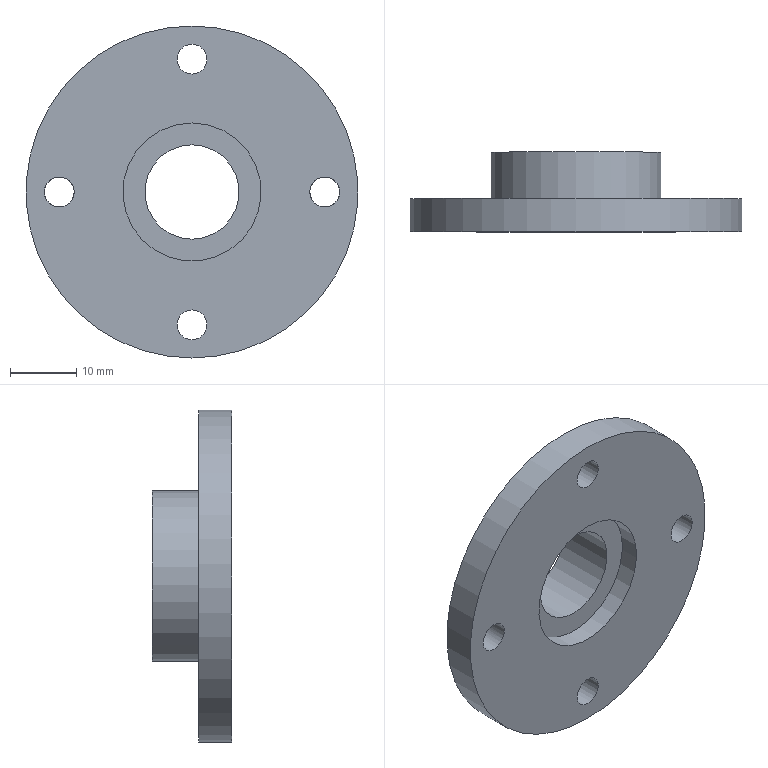Component | NX | END_CAP | 1 solid | 12 faces | box 50 x 12 x 50 mm | volume 10669 mm3 | cylinder 8 | plane 4 | commonest cylinder face diameters 4.5 x4 14.2 x1 20.8 x1 50 x1 25.641 x1
STEP:
#1=CARTESIAN_POINT('',(0.,0.,0.));
#2=DIRECTION('',(0.,0.,1.));
#3=DIRECTION('',(1.,0.,0.));
#4=AXIS2_PLACEMENT_3D('',#1,#2,#3);
#5=CARTESIAN_POINT('',(0.,64.,92.2));
#6=VERTEX_POINT('',#5);
#7=CARTESIAN_POINT('',(0.,64.,85.1));
#8=DIRECTION('',(0.,1.,0.));
#9=DIRECTION('',(0.,0.,1.));
#10=AXIS2_PLACEMENT_3D('',#7,#8,#9);
#11=CIRCLE('',#10,7.1);
#12=CARTESIAN_POINT('',(12.821,64.,85.1));
#13=DIRECTION('',(0.,-1.,0.));
#14=DIRECTION('',(0.,0.,-1.));
#15=AXIS2_PLACEMENT_3D('',#12,#13,#14);
#16=PLANE('',#15);
#17=CARTESIAN_POINT('',(-7.1,-12.821));
#18=CARTESIAN_POINT('',(-7.1,-0.523));
#19=CARTESIAN_POINT('',(3.55,-6.672));
#20=CARTESIAN_POINT('',(14.2,-12.821));
#21=CARTESIAN_POINT('',(3.55,-18.969));
#22=CARTESIAN_POINT('',(-7.1,-25.118));
#23=CARTESIAN_POINT('',(-7.1,-12.821));
#24=(BOUNDED_CURVE()B_SPLINE_CURVE(2,(#17,#18,#19,#20,#21,#22,#23),.UNSPECIFIED.,.T.,.F.)B_SPLINE_CURVE_WITH_KNOTS((1,2,2,2,2,1),(-2.094,0.,2.094,4.189,6.283,8.378),.UNSPECIFIED.)CURVE()GEOMETRIC_REPRESENTATION_ITEM()RATIONAL_B_SPLINE_CURVE((1.,0.5,1.,0.5,1.,0.5,1.))REPRESENTATION_ITEM(''));
#25=(GEOMETRIC_REPRESENTATION_CONTEXT(2)PARAMETRIC_REPRESENTATION_CONTEXT()REPRESENTATION_CONTEXT('',''));
#26=DEFINITIONAL_REPRESENTATION('',(#24),#25);
#27=PCURVE('',#16,#26);
#28=CARTESIAN_POINT('',(0.,52.,85.1));
#29=DIRECTION('',(0.,1.,0.));
#30=DIRECTION('',(0.,0.,1.));
#31=AXIS2_PLACEMENT_3D('',#28,#29,#30);
#32=CYLINDRICAL_SURFACE('',#31,7.1);
#33=CARTESIAN_POINT('',(0.,12.));
#34=DIRECTION('',(1.,0.));
#35=VECTOR('',#34,1.);
#36=LINE('',#33,#35);
#37=(GEOMETRIC_REPRESENTATION_CONTEXT(2)PARAMETRIC_REPRESENTATION_CONTEXT()REPRESENTATION_CONTEXT('',''));
#38=DEFINITIONAL_REPRESENTATION('',(#36),#37);
#39=PCURVE('',#32,#38);
#40=SURFACE_CURVE('',#11,(#27,#39),.PCURVE_S1.);
#41=EDGE_CURVE('',#6,#6,#40,.T.);
#42=ORIENTED_EDGE('',*,*,#41,.F.);
#43=EDGE_LOOP('',(#42));
#44=FACE_BOUND('',#43,.T.);
#45=CARTESIAN_POINT('',(0.,64.,97.921));
#46=VERTEX_POINT('',#45);
#47=CARTESIAN_POINT('',(0.,64.,85.1));
#48=DIRECTION('',(0.,1.,0.));
#49=DIRECTION('',(0.,0.,1.));
#50=AXIS2_PLACEMENT_3D('',#47,#48,#49);
#51=CIRCLE('',#50,12.821);
#52=CARTESIAN_POINT('',(-12.821,-12.821));
#53=CARTESIAN_POINT('',(-12.821,9.385));
#54=CARTESIAN_POINT('',(6.41,-1.718));
#55=CARTESIAN_POINT('',(25.641,-12.821));
#56=CARTESIAN_POINT('',(6.41,-23.923));
#57=CARTESIAN_POINT('',(-12.821,-35.026));
#58=CARTESIAN_POINT('',(-12.821,-12.821));
#59=(BOUNDED_CURVE()B_SPLINE_CURVE(2,(#52,#53,#54,#55,#56,#57,#58),.UNSPECIFIED.,.T.,.F.)B_SPLINE_CURVE_WITH_KNOTS((1,2,2,2,2,1),(-2.094,0.,2.094,4.189,6.283,8.378),.UNSPECIFIED.)CURVE()GEOMETRIC_REPRESENTATION_ITEM()RATIONAL_B_SPLINE_CURVE((1.,0.5,1.,0.5,1.,0.5,1.))REPRESENTATION_ITEM(''));
#60=(GEOMETRIC_REPRESENTATION_CONTEXT(2)PARAMETRIC_REPRESENTATION_CONTEXT()REPRESENTATION_CONTEXT('',''));
#61=DEFINITIONAL_REPRESENTATION('',(#59),#60);
#62=PCURVE('',#16,#61);
#63=CARTESIAN_POINT('',(0.,52.,85.1));
#64=DIRECTION('',(0.,1.,0.));
#65=DIRECTION('',(0.,0.,1.));
#66=AXIS2_PLACEMENT_3D('',#63,#64,#65);
#67=CYLINDRICAL_SURFACE('',#66,12.821);
#68=CARTESIAN_POINT('',(0.,12.));
#69=DIRECTION('',(1.,0.));
#70=VECTOR('',#69,1.);
#71=LINE('',#68,#70);
#72=(GEOMETRIC_REPRESENTATION_CONTEXT(2)PARAMETRIC_REPRESENTATION_CONTEXT()REPRESENTATION_CONTEXT('',''));
#73=DEFINITIONAL_REPRESENTATION('',(#71),#72);
#74=PCURVE('',#67,#73);
#75=SURFACE_CURVE('',#51,(#62,#74),.PCURVE_S1.);
#76=EDGE_CURVE('',#46,#46,#75,.T.);
#77=ORIENTED_EDGE('',*,*,#76,.T.);
#78=EDGE_LOOP('',(#77));
#79=FACE_BOUND('',#78,.T.);
#80=ADVANCED_FACE('',(#44,#79),#16,.F.);
#81=CARTESIAN_POINT('',(0.,55.,92.2));
#82=VERTEX_POINT('',#81);
#83=CARTESIAN_POINT('',(0.,55.,85.1));
#84=DIRECTION('',(0.,1.,0.));
#85=DIRECTION('',(0.,0.,1.));
#86=AXIS2_PLACEMENT_3D('',#83,#84,#85);
#87=CIRCLE('',#86,7.1);
#88=CARTESIAN_POINT('',(0.,3.));
#89=DIRECTION('',(1.,0.));
#90=VECTOR('',#89,1.);
#91=LINE('',#88,#90);
#92=(GEOMETRIC_REPRESENTATION_CONTEXT(2)PARAMETRIC_REPRESENTATION_CONTEXT()REPRESENTATION_CONTEXT('',''));
#93=DEFINITIONAL_REPRESENTATION('',(#91),#92);
#94=PCURVE('',#32,#93);
#95=CARTESIAN_POINT('',(7.1,55.,85.1));
#96=DIRECTION('',(0.,1.,0.));
#97=DIRECTION('',(0.,0.,1.));
#98=AXIS2_PLACEMENT_3D('',#95,#96,#97);
#99=PLANE('',#98);
#100=CARTESIAN_POINT('',(0.,-7.1));
#101=DIRECTION('',(1.,0.));
#102=AXIS2_PLACEMENT_2D('',#100,#101);
#103=CIRCLE('',#102,7.1);
#104=(GEOMETRIC_REPRESENTATION_CONTEXT(2)PARAMETRIC_REPRESENTATION_CONTEXT()REPRESENTATION_CONTEXT('',''));
#105=DEFINITIONAL_REPRESENTATION('',(#103),#104);
#106=PCURVE('',#99,#105);
#107=SURFACE_CURVE('',#87,(#94,#106),.PCURVE_S1.);
#108=EDGE_CURVE('',#82,#82,#107,.T.);
#109=ORIENTED_EDGE('',*,*,#108,.T.);
#110=CARTESIAN_POINT('',(0.,55.,92.2));
#111=CARTESIAN_POINT('',(0.,64.,92.2));
#112=B_SPLINE_CURVE_WITH_KNOTS('',1,(#110,#111),.UNSPECIFIED.,.F.,.F.,(2,2),(3.,12.),.PIECEWISE_BEZIER_KNOTS.);
#113=CARTESIAN_POINT('',(6.283,0.));
#114=DIRECTION('',(0.,1.));
#115=VECTOR('',#114,1.);
#116=LINE('',#113,#115);
#117=(GEOMETRIC_REPRESENTATION_CONTEXT(2)PARAMETRIC_REPRESENTATION_CONTEXT()REPRESENTATION_CONTEXT('',''));
#118=DEFINITIONAL_REPRESENTATION('',(#116),#117);
#119=PCURVE('',#32,#118);
#120=CARTESIAN_POINT('',(0.,0.));
#121=DIRECTION('',(0.,1.));
#122=VECTOR('',#121,1.);
#123=LINE('',#120,#122);
#124=(GEOMETRIC_REPRESENTATION_CONTEXT(2)PARAMETRIC_REPRESENTATION_CONTEXT()REPRESENTATION_CONTEXT('',''));
#125=DEFINITIONAL_REPRESENTATION('',(#123),#124);
#126=PCURVE('',#32,#125);
#127=SEAM_CURVE('',#112,(#119,#126),.PCURVE_S1.);
#128=EDGE_CURVE('',#82,#6,#127,.T.);
#129=ORIENTED_EDGE('',*,*,#128,.T.);
#130=ORIENTED_EDGE('',*,*,#41,.F.);
#131=ORIENTED_EDGE('',*,*,#128,.F.);
#132=EDGE_LOOP('',(#109,#129,#130,#131));
#133=FACE_BOUND('',#132,.F.);
#134=ADVANCED_FACE('',(#133),#32,.F.);
#135=CARTESIAN_POINT('',(0.,55.,95.5));
#136=VERTEX_POINT('',#135);
#137=CARTESIAN_POINT('',(0.,55.,85.1));
#138=DIRECTION('',(0.,1.,0.));
#139=DIRECTION('',(0.,0.,1.));
#140=AXIS2_PLACEMENT_3D('',#137,#138,#139);
#141=CIRCLE('',#140,10.4);
#142=CARTESIAN_POINT('',(0.,-7.1));
#143=DIRECTION('',(1.,0.));
#144=AXIS2_PLACEMENT_2D('',#142,#143);
#145=CIRCLE('',#144,10.4);
#146=(GEOMETRIC_REPRESENTATION_CONTEXT(2)PARAMETRIC_REPRESENTATION_CONTEXT()REPRESENTATION_CONTEXT('',''));
#147=DEFINITIONAL_REPRESENTATION('',(#145),#146);
#148=PCURVE('',#99,#147);
#149=CARTESIAN_POINT('',(0.,52.,85.1));
#150=DIRECTION('',(0.,1.,0.));
#151=DIRECTION('',(0.,0.,1.));
#152=AXIS2_PLACEMENT_3D('',#149,#150,#151);
#153=CYLINDRICAL_SURFACE('',#152,10.4);
#154=CARTESIAN_POINT('',(0.,3.));
#155=DIRECTION('',(1.,0.));
#156=VECTOR('',#155,1.);
#157=LINE('',#154,#156);
#158=(GEOMETRIC_REPRESENTATION_CONTEXT(2)PARAMETRIC_REPRESENTATION_CONTEXT()REPRESENTATION_CONTEXT('',''));
#159=DEFINITIONAL_REPRESENTATION('',(#157),#158);
#160=PCURVE('',#153,#159);
#161=SURFACE_CURVE('',#141,(#148,#160),.PCURVE_S1.);
#162=EDGE_CURVE('',#136,#136,#161,.T.);
#163=ORIENTED_EDGE('',*,*,#162,.F.);
#164=EDGE_LOOP('',(#163));
#165=FACE_BOUND('',#164,.T.);
#166=ORIENTED_EDGE('',*,*,#108,.T.);
#167=EDGE_LOOP('',(#166));
#168=FACE_BOUND('',#167,.T.);
#169=ADVANCED_FACE('',(#165,#168),#99,.F.);
#170=CARTESIAN_POINT('',(0.,52.,95.5));
#171=VERTEX_POINT('',#170);
#172=CARTESIAN_POINT('',(0.,52.,85.1));
#173=DIRECTION('',(0.,1.,0.));
#174=DIRECTION('',(0.,0.,1.));
#175=AXIS2_PLACEMENT_3D('',#172,#173,#174);
#176=CIRCLE('',#175,10.4);
#177=CARTESIAN_POINT('',(0.,0.));
#178=DIRECTION('',(1.,0.));
#179=VECTOR('',#178,1.);
#180=LINE('',#177,#179);
#181=(GEOMETRIC_REPRESENTATION_CONTEXT(2)PARAMETRIC_REPRESENTATION_CONTEXT()REPRESENTATION_CONTEXT('',''));
#182=DEFINITIONAL_REPRESENTATION('',(#180),#181);
#183=PCURVE('',#153,#182);
#184=CARTESIAN_POINT('',(10.4,52.,85.1));
#185=DIRECTION('',(0.,1.,0.));
#186=DIRECTION('',(0.,0.,1.));
#187=AXIS2_PLACEMENT_3D('',#184,#185,#186);
#188=PLANE('',#187);
#189=CARTESIAN_POINT('',(0.,-10.4));
#190=DIRECTION('',(1.,0.));
#191=AXIS2_PLACEMENT_2D('',#189,#190);
#192=CIRCLE('',#191,10.4);
#193=(GEOMETRIC_REPRESENTATION_CONTEXT(2)PARAMETRIC_REPRESENTATION_CONTEXT()REPRESENTATION_CONTEXT('',''));
#194=DEFINITIONAL_REPRESENTATION('',(#192),#193);
#195=PCURVE('',#188,#194);
#196=SURFACE_CURVE('',#176,(#183,#195),.PCURVE_S1.);
#197=EDGE_CURVE('',#171,#171,#196,.T.);
#198=ORIENTED_EDGE('',*,*,#197,.T.);
#199=CARTESIAN_POINT('',(0.,52.,95.5));
#200=CARTESIAN_POINT('',(0.,55.,95.5));
#201=B_SPLINE_CURVE_WITH_KNOTS('',1,(#199,#200),.UNSPECIFIED.,.F.,.F.,(2,2),(0.,3.),.PIECEWISE_BEZIER_KNOTS.);
#202=CARTESIAN_POINT('',(6.283,0.));
#203=DIRECTION('',(0.,1.));
#204=VECTOR('',#203,1.);
#205=LINE('',#202,#204);
#206=(GEOMETRIC_REPRESENTATION_CONTEXT(2)PARAMETRIC_REPRESENTATION_CONTEXT()REPRESENTATION_CONTEXT('',''));
#207=DEFINITIONAL_REPRESENTATION('',(#205),#206);
#208=PCURVE('',#153,#207);
#209=CARTESIAN_POINT('',(0.,0.));
#210=DIRECTION('',(0.,1.));
#211=VECTOR('',#210,1.);
#212=LINE('',#209,#211);
#213=(GEOMETRIC_REPRESENTATION_CONTEXT(2)PARAMETRIC_REPRESENTATION_CONTEXT()REPRESENTATION_CONTEXT('',''));
#214=DEFINITIONAL_REPRESENTATION('',(#212),#213);
#215=PCURVE('',#153,#214);
#216=SEAM_CURVE('',#201,(#208,#215),.PCURVE_S1.);
#217=EDGE_CURVE('',#171,#136,#216,.T.);
#218=ORIENTED_EDGE('',*,*,#217,.T.);
#219=ORIENTED_EDGE('',*,*,#162,.F.);
#220=ORIENTED_EDGE('',*,*,#217,.F.);
#221=EDGE_LOOP('',(#198,#218,#219,#220));
#222=FACE_BOUND('',#221,.F.);
#223=ADVANCED_FACE('',(#222),#153,.F.);
#224=CARTESIAN_POINT('',(20.,52.,87.35));
#225=VERTEX_POINT('',#224);
#226=CARTESIAN_POINT('',(20.,52.,85.1));
#227=DIRECTION('',(0.,1.,0.));
#228=DIRECTION('',(0.,0.,1.));
#229=AXIS2_PLACEMENT_3D('',#226,#227,#228);
#230=CIRCLE('',#229,2.25);
#231=CARTESIAN_POINT('',(0.,9.6));
#232=DIRECTION('',(1.,0.));
#233=AXIS2_PLACEMENT_2D('',#231,#232);
#234=CIRCLE('',#233,2.25);
#235=(GEOMETRIC_REPRESENTATION_CONTEXT(2)PARAMETRIC_REPRESENTATION_CONTEXT()REPRESENTATION_CONTEXT('',''));
#236=DEFINITIONAL_REPRESENTATION('',(#234),#235);
#237=PCURVE('',#188,#236);
#238=CARTESIAN_POINT('',(20.,47.,85.1));
#239=DIRECTION('',(0.,1.,0.));
#240=DIRECTION('',(0.,0.,1.));
#241=AXIS2_PLACEMENT_3D('',#238,#239,#240);
#242=CYLINDRICAL_SURFACE('',#241,2.25);
#243=CARTESIAN_POINT('',(0.,5.));
#244=DIRECTION('',(1.,0.));
#245=VECTOR('',#244,1.);
#246=LINE('',#243,#245);
#247=(GEOMETRIC_REPRESENTATION_CONTEXT(2)PARAMETRIC_REPRESENTATION_CONTEXT()REPRESENTATION_CONTEXT('',''));
#248=DEFINITIONAL_REPRESENTATION('',(#246),#247);
#249=PCURVE('',#242,#248);
#250=SURFACE_CURVE('',#230,(#237,#249),.PCURVE_S1.);
#251=EDGE_CURVE('',#225,#225,#250,.T.);
#252=ORIENTED_EDGE('',*,*,#251,.T.);
#253=EDGE_LOOP('',(#252));
#254=FACE_BOUND('',#253,.T.);
#255=CARTESIAN_POINT('',(0.,52.,67.35));
#256=VERTEX_POINT('',#255);
#257=CARTESIAN_POINT('',(0.,52.,65.1));
#258=DIRECTION('',(0.,1.,0.));
#259=DIRECTION('',(0.,0.,1.));
#260=AXIS2_PLACEMENT_3D('',#257,#258,#259);
#261=CIRCLE('',#260,2.25);
#262=CARTESIAN_POINT('',(-20.,-10.4));
#263=DIRECTION('',(1.,0.));
#264=AXIS2_PLACEMENT_2D('',#262,#263);
#265=CIRCLE('',#264,2.25);
#266=(GEOMETRIC_REPRESENTATION_CONTEXT(2)PARAMETRIC_REPRESENTATION_CONTEXT()REPRESENTATION_CONTEXT('',''));
#267=DEFINITIONAL_REPRESENTATION('',(#265),#266);
#268=PCURVE('',#188,#267);
#269=CARTESIAN_POINT('',(0.,47.,65.1));
#270=DIRECTION('',(0.,1.,0.));
#271=DIRECTION('',(0.,0.,1.));
#272=AXIS2_PLACEMENT_3D('',#269,#270,#271);
#273=CYLINDRICAL_SURFACE('',#272,2.25);
#274=CARTESIAN_POINT('',(0.,5.));
#275=DIRECTION('',(1.,0.));
#276=VECTOR('',#275,1.);
#277=LINE('',#274,#276);
#278=(GEOMETRIC_REPRESENTATION_CONTEXT(2)PARAMETRIC_REPRESENTATION_CONTEXT()REPRESENTATION_CONTEXT('',''));
#279=DEFINITIONAL_REPRESENTATION('',(#277),#278);
#280=PCURVE('',#273,#279);
#281=SURFACE_CURVE('',#261,(#268,#280),.PCURVE_S1.);
#282=EDGE_CURVE('',#256,#256,#281,.T.);
#283=ORIENTED_EDGE('',*,*,#282,.T.);
#284=EDGE_LOOP('',(#283));
#285=FACE_BOUND('',#284,.T.);
#286=CARTESIAN_POINT('',(-20.,52.,87.35));
#287=VERTEX_POINT('',#286);
#288=CARTESIAN_POINT('',(-20.,52.,85.1));
#289=DIRECTION('',(0.,1.,0.));
#290=DIRECTION('',(0.,0.,1.));
#291=AXIS2_PLACEMENT_3D('',#288,#289,#290);
#292=CIRCLE('',#291,2.25);
#293=CARTESIAN_POINT('',(0.,-30.4));
#294=DIRECTION('',(1.,0.));
#295=AXIS2_PLACEMENT_2D('',#293,#294);
#296=CIRCLE('',#295,2.25);
#297=(GEOMETRIC_REPRESENTATION_CONTEXT(2)PARAMETRIC_REPRESENTATION_CONTEXT()REPRESENTATION_CONTEXT('',''));
#298=DEFINITIONAL_REPRESENTATION('',(#296),#297);
#299=PCURVE('',#188,#298);
#300=CARTESIAN_POINT('',(-20.,47.,85.1));
#301=DIRECTION('',(0.,1.,0.));
#302=DIRECTION('',(0.,0.,1.));
#303=AXIS2_PLACEMENT_3D('',#300,#301,#302);
#304=CYLINDRICAL_SURFACE('',#303,2.25);
#305=CARTESIAN_POINT('',(0.,5.));
#306=DIRECTION('',(1.,0.));
#307=VECTOR('',#306,1.);
#308=LINE('',#305,#307);
#309=(GEOMETRIC_REPRESENTATION_CONTEXT(2)PARAMETRIC_REPRESENTATION_CONTEXT()REPRESENTATION_CONTEXT('',''));
#310=DEFINITIONAL_REPRESENTATION('',(#308),#309);
#311=PCURVE('',#304,#310);
#312=SURFACE_CURVE('',#292,(#299,#311),.PCURVE_S1.);
#313=EDGE_CURVE('',#287,#287,#312,.T.);
#314=ORIENTED_EDGE('',*,*,#313,.T.);
#315=EDGE_LOOP('',(#314));
#316=FACE_BOUND('',#315,.T.);
#317=CARTESIAN_POINT('',(0.,52.,107.35));
#318=VERTEX_POINT('',#317);
#319=CARTESIAN_POINT('',(0.,52.,105.1));
#320=DIRECTION('',(0.,1.,0.));
#321=DIRECTION('',(0.,0.,1.));
#322=AXIS2_PLACEMENT_3D('',#319,#320,#321);
#323=CIRCLE('',#322,2.25);
#324=CARTESIAN_POINT('',(20.,-10.4));
#325=DIRECTION('',(1.,0.));
#326=AXIS2_PLACEMENT_2D('',#324,#325);
#327=CIRCLE('',#326,2.25);
#328=(GEOMETRIC_REPRESENTATION_CONTEXT(2)PARAMETRIC_REPRESENTATION_CONTEXT()REPRESENTATION_CONTEXT('',''));
#329=DEFINITIONAL_REPRESENTATION('',(#327),#328);
#330=PCURVE('',#188,#329);
#331=CARTESIAN_POINT('',(0.,47.,105.1));
#332=DIRECTION('',(0.,1.,0.));
#333=DIRECTION('',(0.,0.,1.));
#334=AXIS2_PLACEMENT_3D('',#331,#332,#333);
#335=CYLINDRICAL_SURFACE('',#334,2.25);
#336=CARTESIAN_POINT('',(0.,5.));
#337=DIRECTION('',(1.,0.));
#338=VECTOR('',#337,1.);
#339=LINE('',#336,#338);
#340=(GEOMETRIC_REPRESENTATION_CONTEXT(2)PARAMETRIC_REPRESENTATION_CONTEXT()REPRESENTATION_CONTEXT('',''));
#341=DEFINITIONAL_REPRESENTATION('',(#339),#340);
#342=PCURVE('',#335,#341);
#343=SURFACE_CURVE('',#323,(#330,#342),.PCURVE_S1.);
#344=EDGE_CURVE('',#318,#318,#343,.T.);
#345=ORIENTED_EDGE('',*,*,#344,.T.);
#346=EDGE_LOOP('',(#345));
#347=FACE_BOUND('',#346,.T.);
#348=CARTESIAN_POINT('',(0.,52.,110.1));
#349=VERTEX_POINT('',#348);
#350=CARTESIAN_POINT('',(0.,52.,85.1));
#351=DIRECTION('',(0.,1.,0.));
#352=DIRECTION('',(0.,0.,1.));
#353=AXIS2_PLACEMENT_3D('',#350,#351,#352);
#354=CIRCLE('',#353,25.);
#355=CARTESIAN_POINT('',(0.,-10.4));
#356=DIRECTION('',(1.,0.));
#357=AXIS2_PLACEMENT_2D('',#355,#356);
#358=CIRCLE('',#357,25.);
#359=(GEOMETRIC_REPRESENTATION_CONTEXT(2)PARAMETRIC_REPRESENTATION_CONTEXT()REPRESENTATION_CONTEXT('',''));
#360=DEFINITIONAL_REPRESENTATION('',(#358),#359);
#361=PCURVE('',#188,#360);
#362=CARTESIAN_POINT('',(0.,52.,85.1));
#363=DIRECTION('',(0.,1.,0.));
#364=DIRECTION('',(0.,0.,1.));
#365=AXIS2_PLACEMENT_3D('',#362,#363,#364);
#366=CYLINDRICAL_SURFACE('',#365,25.);
#367=CARTESIAN_POINT('',(0.,0.));
#368=DIRECTION('',(1.,0.));
#369=VECTOR('',#368,1.);
#370=LINE('',#367,#369);
#371=(GEOMETRIC_REPRESENTATION_CONTEXT(2)PARAMETRIC_REPRESENTATION_CONTEXT()REPRESENTATION_CONTEXT('',''));
#372=DEFINITIONAL_REPRESENTATION('',(#370),#371);
#373=PCURVE('',#366,#372);
#374=SURFACE_CURVE('',#354,(#361,#373),.PCURVE_S1.);
#375=EDGE_CURVE('',#349,#349,#374,.T.);
#376=ORIENTED_EDGE('',*,*,#375,.F.);
#377=EDGE_LOOP('',(#376));
#378=FACE_BOUND('',#377,.T.);
#379=ORIENTED_EDGE('',*,*,#197,.T.);
#380=EDGE_LOOP('',(#379));
#381=FACE_BOUND('',#380,.T.);
#382=ADVANCED_FACE('',(#254,#285,#316,#347,#378,#381),#188,.F.);
#383=CARTESIAN_POINT('',(0.,57.,110.1));
#384=VERTEX_POINT('',#383);
#385=CARTESIAN_POINT('',(0.,57.,85.1));
#386=DIRECTION('',(0.,1.,0.));
#387=DIRECTION('',(0.,0.,1.));
#388=AXIS2_PLACEMENT_3D('',#385,#386,#387);
#389=CIRCLE('',#388,25.);
#390=CARTESIAN_POINT('',(0.,5.));
#391=DIRECTION('',(1.,0.));
#392=VECTOR('',#391,1.);
#393=LINE('',#390,#392);
#394=(GEOMETRIC_REPRESENTATION_CONTEXT(2)PARAMETRIC_REPRESENTATION_CONTEXT()REPRESENTATION_CONTEXT('',''));
#395=DEFINITIONAL_REPRESENTATION('',(#393),#394);
#396=PCURVE('',#366,#395);
#397=CARTESIAN_POINT('',(25.,57.,85.1));
#398=DIRECTION('',(0.,-1.,0.));
#399=DIRECTION('',(0.,0.,-1.));
#400=AXIS2_PLACEMENT_3D('',#397,#398,#399);
#401=PLANE('',#400);
#402=CARTESIAN_POINT('',(-25.,-25.));
#403=CARTESIAN_POINT('',(-25.,18.301));
#404=CARTESIAN_POINT('',(12.5,-3.349));
#405=CARTESIAN_POINT('',(50.,-25.));
#406=CARTESIAN_POINT('',(12.5,-46.651));
#407=CARTESIAN_POINT('',(-25.,-68.301));
#408=CARTESIAN_POINT('',(-25.,-25.));
#409=(BOUNDED_CURVE()B_SPLINE_CURVE(2,(#402,#403,#404,#405,#406,#407,#408),.UNSPECIFIED.,.T.,.F.)B_SPLINE_CURVE_WITH_KNOTS((1,2,2,2,2,1),(-2.094,0.,2.094,4.189,6.283,8.378),.UNSPECIFIED.)CURVE()GEOMETRIC_REPRESENTATION_ITEM()RATIONAL_B_SPLINE_CURVE((1.,0.5,1.,0.5,1.,0.5,1.))REPRESENTATION_ITEM(''));
#410=(GEOMETRIC_REPRESENTATION_CONTEXT(2)PARAMETRIC_REPRESENTATION_CONTEXT()REPRESENTATION_CONTEXT('',''));
#411=DEFINITIONAL_REPRESENTATION('',(#409),#410);
#412=PCURVE('',#401,#411);
#413=SURFACE_CURVE('',#389,(#396,#412),.PCURVE_S1.);
#414=EDGE_CURVE('',#384,#384,#413,.T.);
#415=ORIENTED_EDGE('',*,*,#414,.F.);
#416=CARTESIAN_POINT('',(0.,52.,110.1));
#417=CARTESIAN_POINT('',(0.,57.,110.1));
#418=B_SPLINE_CURVE_WITH_KNOTS('',1,(#416,#417),.UNSPECIFIED.,.F.,.F.,(2,2),(0.,5.),.PIECEWISE_BEZIER_KNOTS.);
#419=CARTESIAN_POINT('',(0.,0.));
#420=DIRECTION('',(0.,1.));
#421=VECTOR('',#420,1.);
#422=LINE('',#419,#421);
#423=(GEOMETRIC_REPRESENTATION_CONTEXT(2)PARAMETRIC_REPRESENTATION_CONTEXT()REPRESENTATION_CONTEXT('',''));
#424=DEFINITIONAL_REPRESENTATION('',(#422),#423);
#425=PCURVE('',#366,#424);
#426=CARTESIAN_POINT('',(6.283,0.));
#427=DIRECTION('',(0.,1.));
#428=VECTOR('',#427,1.);
#429=LINE('',#426,#428);
#430=(GEOMETRIC_REPRESENTATION_CONTEXT(2)PARAMETRIC_REPRESENTATION_CONTEXT()REPRESENTATION_CONTEXT('',''));
#431=DEFINITIONAL_REPRESENTATION('',(#429),#430);
#432=PCURVE('',#366,#431);
#433=SEAM_CURVE('',#418,(#425,#432),.PCURVE_S1.);
#434=EDGE_CURVE('',#349,#384,#433,.T.);
#435=ORIENTED_EDGE('',*,*,#434,.F.);
#436=ORIENTED_EDGE('',*,*,#375,.T.);
#437=ORIENTED_EDGE('',*,*,#434,.T.);
#438=EDGE_LOOP('',(#415,#435,#436,#437));
#439=FACE_BOUND('',#438,.T.);
#440=ADVANCED_FACE('',(#439),#366,.T.);
#441=CARTESIAN_POINT('',(17.75,57.,85.1));
#442=VERTEX_POINT('',#441);
#443=CARTESIAN_POINT('',(20.,57.,87.35));
#444=VERTEX_POINT('',#443);
#445=CARTESIAN_POINT('',(20.,57.,85.1));
#446=DIRECTION('',(0.,1.,0.));
#447=DIRECTION('',(-1.,0.,0.));
#448=AXIS2_PLACEMENT_3D('',#445,#446,#447);
#449=CIRCLE('',#448,2.25);
#450=CARTESIAN_POINT('',(0.,-7.25));
#451=CARTESIAN_POINT('',(-3.897,-7.25));
#452=CARTESIAN_POINT('',(-1.949,-3.875));
#453=CARTESIAN_POINT('',(-0.,-0.5));
#454=CARTESIAN_POINT('',(1.949,-3.875));
#455=CARTESIAN_POINT('',(3.897,-7.25));
#456=CARTESIAN_POINT('',(0.,-7.25));
#457=(BOUNDED_CURVE()B_SPLINE_CURVE(2,(#450,#451,#452,#453,#454,#455,#456),.UNSPECIFIED.,.T.,.F.)B_SPLINE_CURVE_WITH_KNOTS((1,2,2,2,2,1),(-2.094,0.,2.094,4.189,6.283,8.378),.UNSPECIFIED.)CURVE()GEOMETRIC_REPRESENTATION_ITEM()RATIONAL_B_SPLINE_CURVE((1.,0.5,1.,0.5,1.,0.5,1.))REPRESENTATION_ITEM(''));
#458=(GEOMETRIC_REPRESENTATION_CONTEXT(2)PARAMETRIC_REPRESENTATION_CONTEXT()REPRESENTATION_CONTEXT('',''));
#459=DEFINITIONAL_REPRESENTATION('',(#457),#458);
#460=PCURVE('',#401,#459);
#461=CARTESIAN_POINT('',(4.712,10.));
#462=DIRECTION('',(1.,0.));
#463=VECTOR('',#462,1.);
#464=LINE('',#461,#463);
#465=(GEOMETRIC_REPRESENTATION_CONTEXT(2)PARAMETRIC_REPRESENTATION_CONTEXT()REPRESENTATION_CONTEXT('',''));
#466=DEFINITIONAL_REPRESENTATION('',(#464),#465);
#467=PCURVE('',#242,#466);
#468=SURFACE_CURVE('',#449,(#460,#467),.PCURVE_S1.);
#469=EDGE_CURVE('',#442,#444,#468,.T.);
#470=ORIENTED_EDGE('',*,*,#469,.F.);
#471=CARTESIAN_POINT('',(20.,57.,85.1));
#472=DIRECTION('',(0.,1.,0.));
#473=DIRECTION('',(-1.,0.,0.));
#474=AXIS2_PLACEMENT_3D('',#471,#472,#473);
#475=CIRCLE('',#474,2.25);
#476=CARTESIAN_POINT('',(0.,-7.25));
#477=CARTESIAN_POINT('',(-3.897,-7.25));
#478=CARTESIAN_POINT('',(-1.949,-3.875));
#479=CARTESIAN_POINT('',(-0.,-0.5));
#480=CARTESIAN_POINT('',(1.949,-3.875));
#481=CARTESIAN_POINT('',(3.897,-7.25));
#482=CARTESIAN_POINT('',(0.,-7.25));
#483=(BOUNDED_CURVE()B_SPLINE_CURVE(2,(#476,#477,#478,#479,#480,#481,#482),.UNSPECIFIED.,.T.,.F.)B_SPLINE_CURVE_WITH_KNOTS((1,2,2,2,2,1),(-2.094,0.,2.094,4.189,6.283,8.378),.UNSPECIFIED.)CURVE()GEOMETRIC_REPRESENTATION_ITEM()RATIONAL_B_SPLINE_CURVE((1.,0.5,1.,0.5,1.,0.5,1.))REPRESENTATION_ITEM(''));
#484=(GEOMETRIC_REPRESENTATION_CONTEXT(2)PARAMETRIC_REPRESENTATION_CONTEXT()REPRESENTATION_CONTEXT('',''));
#485=DEFINITIONAL_REPRESENTATION('',(#483),#484);
#486=PCURVE('',#401,#485);
#487=CARTESIAN_POINT('',(-1.571,10.));
#488=DIRECTION('',(1.,0.));
#489=VECTOR('',#488,1.);
#490=LINE('',#487,#489);
#491=(GEOMETRIC_REPRESENTATION_CONTEXT(2)PARAMETRIC_REPRESENTATION_CONTEXT()REPRESENTATION_CONTEXT('',''));
#492=DEFINITIONAL_REPRESENTATION('',(#490),#491);
#493=PCURVE('',#242,#492);
#494=SURFACE_CURVE('',#475,(#486,#493),.PCURVE_S1.);
#495=EDGE_CURVE('',#444,#442,#494,.T.);
#496=ORIENTED_EDGE('',*,*,#495,.F.);
#497=EDGE_LOOP('',(#470,#496));
#498=FACE_BOUND('',#497,.T.);
#499=CARTESIAN_POINT('',(0.,57.,67.35));
#500=VERTEX_POINT('',#499);
#501=CARTESIAN_POINT('',(0.,57.,65.1));
#502=DIRECTION('',(0.,1.,0.));
#503=DIRECTION('',(0.,0.,1.));
#504=AXIS2_PLACEMENT_3D('',#501,#502,#503);
#505=CIRCLE('',#504,2.25);
#506=CARTESIAN_POINT('',(17.75,-25.));
#507=CARTESIAN_POINT('',(17.75,-21.103));
#508=CARTESIAN_POINT('',(21.125,-23.051));
#509=CARTESIAN_POINT('',(24.5,-25.));
#510=CARTESIAN_POINT('',(21.125,-26.949));
#511=CARTESIAN_POINT('',(17.75,-28.897));
#512=CARTESIAN_POINT('',(17.75,-25.));
#513=(BOUNDED_CURVE()B_SPLINE_CURVE(2,(#506,#507,#508,#509,#510,#511,#512),.UNSPECIFIED.,.T.,.F.)B_SPLINE_CURVE_WITH_KNOTS((1,2,2,2,2,1),(-2.094,0.,2.094,4.189,6.283,8.378),.UNSPECIFIED.)CURVE()GEOMETRIC_REPRESENTATION_ITEM()RATIONAL_B_SPLINE_CURVE((1.,0.5,1.,0.5,1.,0.5,1.))REPRESENTATION_ITEM(''));
#514=(GEOMETRIC_REPRESENTATION_CONTEXT(2)PARAMETRIC_REPRESENTATION_CONTEXT()REPRESENTATION_CONTEXT('',''));
#515=DEFINITIONAL_REPRESENTATION('',(#513),#514);
#516=PCURVE('',#401,#515);
#517=CARTESIAN_POINT('',(0.,10.));
#518=DIRECTION('',(1.,0.));
#519=VECTOR('',#518,1.);
#520=LINE('',#517,#519);
#521=(GEOMETRIC_REPRESENTATION_CONTEXT(2)PARAMETRIC_REPRESENTATION_CONTEXT()REPRESENTATION_CONTEXT('',''));
#522=DEFINITIONAL_REPRESENTATION('',(#520),#521);
#523=PCURVE('',#273,#522);
#524=SURFACE_CURVE('',#505,(#516,#523),.PCURVE_S1.);
#525=EDGE_CURVE('',#500,#500,#524,.T.);
#526=ORIENTED_EDGE('',*,*,#525,.F.);
#527=EDGE_LOOP('',(#526));
#528=FACE_BOUND('',#527,.T.);
#529=CARTESIAN_POINT('',(-17.75,57.,85.1));
#530=VERTEX_POINT('',#529);
#531=CARTESIAN_POINT('',(-20.,57.,87.35));
#532=VERTEX_POINT('',#531);
#533=CARTESIAN_POINT('',(-20.,57.,85.1));
#534=DIRECTION('',(0.,1.,0.));
#535=DIRECTION('',(1.,0.,0.));
#536=AXIS2_PLACEMENT_3D('',#533,#534,#535);
#537=CIRCLE('',#536,2.25);
#538=CARTESIAN_POINT('',(0.,-42.75));
#539=CARTESIAN_POINT('',(3.897,-42.75));
#540=CARTESIAN_POINT('',(1.949,-46.125));
#541=CARTESIAN_POINT('',(0.,-49.5));
#542=CARTESIAN_POINT('',(-1.949,-46.125));
#543=CARTESIAN_POINT('',(-3.897,-42.75));
#544=CARTESIAN_POINT('',(0.,-42.75));
#545=(BOUNDED_CURVE()B_SPLINE_CURVE(2,(#538,#539,#540,#541,#542,#543,#544),.UNSPECIFIED.,.T.,.F.)B_SPLINE_CURVE_WITH_KNOTS((1,2,2,2,2,1),(-2.094,0.,2.094,4.189,6.283,8.378),.UNSPECIFIED.)CURVE()GEOMETRIC_REPRESENTATION_ITEM()RATIONAL_B_SPLINE_CURVE((1.,0.5,1.,0.5,1.,0.5,1.))REPRESENTATION_ITEM(''));
#546=(GEOMETRIC_REPRESENTATION_CONTEXT(2)PARAMETRIC_REPRESENTATION_CONTEXT()REPRESENTATION_CONTEXT('',''));
#547=DEFINITIONAL_REPRESENTATION('',(#545),#546);
#548=PCURVE('',#401,#547);
#549=CARTESIAN_POINT('',(1.571,10.));
#550=DIRECTION('',(1.,0.));
#551=VECTOR('',#550,1.);
#552=LINE('',#549,#551);
#553=(GEOMETRIC_REPRESENTATION_CONTEXT(2)PARAMETRIC_REPRESENTATION_CONTEXT()REPRESENTATION_CONTEXT('',''));
#554=DEFINITIONAL_REPRESENTATION('',(#552),#553);
#555=PCURVE('',#304,#554);
#556=SURFACE_CURVE('',#537,(#548,#555),.PCURVE_S1.);
#557=EDGE_CURVE('',#530,#532,#556,.T.);
#558=ORIENTED_EDGE('',*,*,#557,.F.);
#559=CARTESIAN_POINT('',(-20.,57.,85.1));
#560=DIRECTION('',(0.,1.,0.));
#561=DIRECTION('',(1.,0.,0.));
#562=AXIS2_PLACEMENT_3D('',#559,#560,#561);
#563=CIRCLE('',#562,2.25);
#564=CARTESIAN_POINT('',(0.,-42.75));
#565=CARTESIAN_POINT('',(3.897,-42.75));
#566=CARTESIAN_POINT('',(1.949,-46.125));
#567=CARTESIAN_POINT('',(0.,-49.5));
#568=CARTESIAN_POINT('',(-1.949,-46.125));
#569=CARTESIAN_POINT('',(-3.897,-42.75));
#570=CARTESIAN_POINT('',(0.,-42.75));
#571=(BOUNDED_CURVE()B_SPLINE_CURVE(2,(#564,#565,#566,#567,#568,#569,#570),.UNSPECIFIED.,.T.,.F.)B_SPLINE_CURVE_WITH_KNOTS((1,2,2,2,2,1),(-2.094,0.,2.094,4.189,6.283,8.378),.UNSPECIFIED.)CURVE()GEOMETRIC_REPRESENTATION_ITEM()RATIONAL_B_SPLINE_CURVE((1.,0.5,1.,0.5,1.,0.5,1.))REPRESENTATION_ITEM(''));
#572=(GEOMETRIC_REPRESENTATION_CONTEXT(2)PARAMETRIC_REPRESENTATION_CONTEXT()REPRESENTATION_CONTEXT('',''));
#573=DEFINITIONAL_REPRESENTATION('',(#571),#572);
#574=PCURVE('',#401,#573);
#575=CARTESIAN_POINT('',(-4.712,10.));
#576=DIRECTION('',(1.,0.));
#577=VECTOR('',#576,1.);
#578=LINE('',#575,#577);
#579=(GEOMETRIC_REPRESENTATION_CONTEXT(2)PARAMETRIC_REPRESENTATION_CONTEXT()REPRESENTATION_CONTEXT('',''));
#580=DEFINITIONAL_REPRESENTATION('',(#578),#579);
#581=PCURVE('',#304,#580);
#582=SURFACE_CURVE('',#563,(#574,#581),.PCURVE_S1.);
#583=EDGE_CURVE('',#532,#530,#582,.T.);
#584=ORIENTED_EDGE('',*,*,#583,.F.);
#585=EDGE_LOOP('',(#558,#584));
#586=FACE_BOUND('',#585,.T.);
#587=CARTESIAN_POINT('',(0.,57.,102.85));
#588=VERTEX_POINT('',#587);
#589=CARTESIAN_POINT('',(0.,57.,107.35));
#590=VERTEX_POINT('',#589);
#591=CARTESIAN_POINT('',(0.,57.,105.1));
#592=DIRECTION('',(0.,1.,0.));
#593=DIRECTION('',(0.,0.,-1.));
#594=AXIS2_PLACEMENT_3D('',#591,#592,#593);
#595=CIRCLE('',#594,2.25);
#596=CARTESIAN_POINT('',(-17.75,-25.));
#597=CARTESIAN_POINT('',(-17.75,-28.897));
#598=CARTESIAN_POINT('',(-21.125,-26.949));
#599=CARTESIAN_POINT('',(-24.5,-25.));
#600=CARTESIAN_POINT('',(-21.125,-23.051));
#601=CARTESIAN_POINT('',(-17.75,-21.103));
#602=CARTESIAN_POINT('',(-17.75,-25.));
#603=(BOUNDED_CURVE()B_SPLINE_CURVE(2,(#596,#597,#598,#599,#600,#601,#602),.UNSPECIFIED.,.T.,.F.)B_SPLINE_CURVE_WITH_KNOTS((1,2,2,2,2,1),(-2.094,0.,2.094,4.189,6.283,8.378),.UNSPECIFIED.)CURVE()GEOMETRIC_REPRESENTATION_ITEM()RATIONAL_B_SPLINE_CURVE((1.,0.5,1.,0.5,1.,0.5,1.))REPRESENTATION_ITEM(''));
#604=(GEOMETRIC_REPRESENTATION_CONTEXT(2)PARAMETRIC_REPRESENTATION_CONTEXT()REPRESENTATION_CONTEXT('',''));
#605=DEFINITIONAL_REPRESENTATION('',(#603),#604);
#606=PCURVE('',#401,#605);
#607=CARTESIAN_POINT('',(3.142,10.));
#608=DIRECTION('',(1.,0.));
#609=VECTOR('',#608,1.);
#610=LINE('',#607,#609);
#611=(GEOMETRIC_REPRESENTATION_CONTEXT(2)PARAMETRIC_REPRESENTATION_CONTEXT()REPRESENTATION_CONTEXT('',''));
#612=DEFINITIONAL_REPRESENTATION('',(#610),#611);
#613=PCURVE('',#335,#612);
#614=SURFACE_CURVE('',#595,(#606,#613),.PCURVE_S1.);
#615=EDGE_CURVE('',#588,#590,#614,.T.);
#616=ORIENTED_EDGE('',*,*,#615,.F.);
#617=CARTESIAN_POINT('',(0.,57.,105.1));
#618=DIRECTION('',(0.,1.,0.));
#619=DIRECTION('',(0.,0.,-1.));
#620=AXIS2_PLACEMENT_3D('',#617,#618,#619);
#621=CIRCLE('',#620,2.25);
#622=CARTESIAN_POINT('',(-17.75,-25.));
#623=CARTESIAN_POINT('',(-17.75,-28.897));
#624=CARTESIAN_POINT('',(-21.125,-26.949));
#625=CARTESIAN_POINT('',(-24.5,-25.));
#626=CARTESIAN_POINT('',(-21.125,-23.051));
#627=CARTESIAN_POINT('',(-17.75,-21.103));
#628=CARTESIAN_POINT('',(-17.75,-25.));
#629=(BOUNDED_CURVE()B_SPLINE_CURVE(2,(#622,#623,#624,#625,#626,#627,#628),.UNSPECIFIED.,.T.,.F.)B_SPLINE_CURVE_WITH_KNOTS((1,2,2,2,2,1),(-2.094,0.,2.094,4.189,6.283,8.378),.UNSPECIFIED.)CURVE()GEOMETRIC_REPRESENTATION_ITEM()RATIONAL_B_SPLINE_CURVE((1.,0.5,1.,0.5,1.,0.5,1.))REPRESENTATION_ITEM(''));
#630=(GEOMETRIC_REPRESENTATION_CONTEXT(2)PARAMETRIC_REPRESENTATION_CONTEXT()REPRESENTATION_CONTEXT('',''));
#631=DEFINITIONAL_REPRESENTATION('',(#629),#630);
#632=PCURVE('',#401,#631);
#633=CARTESIAN_POINT('',(-3.142,10.));
#634=DIRECTION('',(1.,0.));
#635=VECTOR('',#634,1.);
#636=LINE('',#633,#635);
#637=(GEOMETRIC_REPRESENTATION_CONTEXT(2)PARAMETRIC_REPRESENTATION_CONTEXT()REPRESENTATION_CONTEXT('',''));
#638=DEFINITIONAL_REPRESENTATION('',(#636),#637);
#639=PCURVE('',#335,#638);
#640=SURFACE_CURVE('',#621,(#632,#639),.PCURVE_S1.);
#641=EDGE_CURVE('',#590,#588,#640,.T.);
#642=ORIENTED_EDGE('',*,*,#641,.F.);
#643=EDGE_LOOP('',(#616,#642));
#644=FACE_BOUND('',#643,.T.);
#645=CARTESIAN_POINT('',(0.,57.,97.921));
#646=VERTEX_POINT('',#645);
#647=CARTESIAN_POINT('',(0.,57.,85.1));
#648=DIRECTION('',(0.,1.,0.));
#649=DIRECTION('',(0.,0.,1.));
#650=AXIS2_PLACEMENT_3D('',#647,#648,#649);
#651=CIRCLE('',#650,12.821);
#652=CARTESIAN_POINT('',(-12.821,-25.));
#653=CARTESIAN_POINT('',(-12.821,-2.794));
#654=CARTESIAN_POINT('',(6.41,-13.897));
#655=CARTESIAN_POINT('',(25.641,-25.));
#656=CARTESIAN_POINT('',(6.41,-36.103));
#657=CARTESIAN_POINT('',(-12.821,-47.206));
#658=CARTESIAN_POINT('',(-12.821,-25.));
#659=(BOUNDED_CURVE()B_SPLINE_CURVE(2,(#652,#653,#654,#655,#656,#657,#658),.UNSPECIFIED.,.T.,.F.)B_SPLINE_CURVE_WITH_KNOTS((1,2,2,2,2,1),(-2.094,0.,2.094,4.189,6.283,8.378),.UNSPECIFIED.)CURVE()GEOMETRIC_REPRESENTATION_ITEM()RATIONAL_B_SPLINE_CURVE((1.,0.5,1.,0.5,1.,0.5,1.))REPRESENTATION_ITEM(''));
#660=(GEOMETRIC_REPRESENTATION_CONTEXT(2)PARAMETRIC_REPRESENTATION_CONTEXT()REPRESENTATION_CONTEXT('',''));
#661=DEFINITIONAL_REPRESENTATION('',(#659),#660);
#662=PCURVE('',#401,#661);
#663=CARTESIAN_POINT('',(0.,5.));
#664=DIRECTION('',(1.,0.));
#665=VECTOR('',#664,1.);
#666=LINE('',#663,#665);
#667=(GEOMETRIC_REPRESENTATION_CONTEXT(2)PARAMETRIC_REPRESENTATION_CONTEXT()REPRESENTATION_CONTEXT('',''));
#668=DEFINITIONAL_REPRESENTATION('',(#666),#667);
#669=PCURVE('',#67,#668);
#670=SURFACE_CURVE('',#651,(#662,#669),.PCURVE_S1.);
#671=EDGE_CURVE('',#646,#646,#670,.T.);
#672=ORIENTED_EDGE('',*,*,#671,.F.);
#673=EDGE_LOOP('',(#672));
#674=FACE_BOUND('',#673,.T.);
#675=ORIENTED_EDGE('',*,*,#414,.T.);
#676=EDGE_LOOP('',(#675));
#677=FACE_BOUND('',#676,.T.);
#678=ADVANCED_FACE('',(#498,#528,#586,#644,#674,#677),#401,.F.);
#679=ORIENTED_EDGE('',*,*,#76,.F.);
#680=CARTESIAN_POINT('',(0.,57.,97.921));
#681=CARTESIAN_POINT('',(0.,64.,97.921));
#682=B_SPLINE_CURVE_WITH_KNOTS('',1,(#680,#681),.UNSPECIFIED.,.F.,.F.,(2,2),(5.,12.),.PIECEWISE_BEZIER_KNOTS.);
#683=CARTESIAN_POINT('',(0.,0.));
#684=DIRECTION('',(0.,1.));
#685=VECTOR('',#684,1.);
#686=LINE('',#683,#685);
#687=(GEOMETRIC_REPRESENTATION_CONTEXT(2)PARAMETRIC_REPRESENTATION_CONTEXT()REPRESENTATION_CONTEXT('',''));
#688=DEFINITIONAL_REPRESENTATION('',(#686),#687);
#689=PCURVE('',#67,#688);
#690=CARTESIAN_POINT('',(6.283,0.));
#691=DIRECTION('',(0.,1.));
#692=VECTOR('',#691,1.);
#693=LINE('',#690,#692);
#694=(GEOMETRIC_REPRESENTATION_CONTEXT(2)PARAMETRIC_REPRESENTATION_CONTEXT()REPRESENTATION_CONTEXT('',''));
#695=DEFINITIONAL_REPRESENTATION('',(#693),#694);
#696=PCURVE('',#67,#695);
#697=SEAM_CURVE('',#682,(#689,#696),.PCURVE_S1.);
#698=EDGE_CURVE('',#646,#46,#697,.T.);
#699=ORIENTED_EDGE('',*,*,#698,.F.);
#700=ORIENTED_EDGE('',*,*,#671,.T.);
#701=ORIENTED_EDGE('',*,*,#698,.T.);
#702=EDGE_LOOP('',(#679,#699,#700,#701));
#703=FACE_BOUND('',#702,.T.);
#704=ADVANCED_FACE('',(#703),#67,.T.);
#705=ORIENTED_EDGE('',*,*,#641,.F.);
#706=CARTESIAN_POINT('',(0.,52.,107.35));
#707=CARTESIAN_POINT('',(0.,57.,107.35));
#708=B_SPLINE_CURVE_WITH_KNOTS('',1,(#706,#707),.UNSPECIFIED.,.F.,.F.,(2,2),(5.,10.),.PIECEWISE_BEZIER_KNOTS.);
#709=CARTESIAN_POINT('',(0.,0.));
#710=DIRECTION('',(0.,1.));
#711=VECTOR('',#710,1.);
#712=LINE('',#709,#711);
#713=(GEOMETRIC_REPRESENTATION_CONTEXT(2)PARAMETRIC_REPRESENTATION_CONTEXT()REPRESENTATION_CONTEXT('',''));
#714=DEFINITIONAL_REPRESENTATION('',(#712),#713);
#715=PCURVE('',#335,#714);
#716=CARTESIAN_POINT('',(6.283,0.));
#717=DIRECTION('',(0.,1.));
#718=VECTOR('',#717,1.);
#719=LINE('',#716,#718);
#720=(GEOMETRIC_REPRESENTATION_CONTEXT(2)PARAMETRIC_REPRESENTATION_CONTEXT()REPRESENTATION_CONTEXT('',''));
#721=DEFINITIONAL_REPRESENTATION('',(#719),#720);
#722=PCURVE('',#335,#721);
#723=SEAM_CURVE('',#708,(#715,#722),.PCURVE_S1.);
#724=EDGE_CURVE('',#318,#590,#723,.T.);
#725=ORIENTED_EDGE('',*,*,#724,.F.);
#726=ORIENTED_EDGE('',*,*,#344,.T.);
#727=ORIENTED_EDGE('',*,*,#724,.T.);
#728=ORIENTED_EDGE('',*,*,#615,.F.);
#729=EDGE_LOOP('',(#705,#725,#726,#727,#728));
#730=FACE_BOUND('',#729,.F.);
#731=ADVANCED_FACE('',(#730),#335,.F.);
#732=ORIENTED_EDGE('',*,*,#583,.F.);
#733=CARTESIAN_POINT('',(-20.,52.,87.35));
#734=CARTESIAN_POINT('',(-20.,57.,87.35));
#735=B_SPLINE_CURVE_WITH_KNOTS('',1,(#733,#734),.UNSPECIFIED.,.F.,.F.,(2,2),(5.,10.),.PIECEWISE_BEZIER_KNOTS.);
#736=CARTESIAN_POINT('',(0.,0.));
#737=DIRECTION('',(0.,1.));
#738=VECTOR('',#737,1.);
#739=LINE('',#736,#738);
#740=(GEOMETRIC_REPRESENTATION_CONTEXT(2)PARAMETRIC_REPRESENTATION_CONTEXT()REPRESENTATION_CONTEXT('',''));
#741=DEFINITIONAL_REPRESENTATION('',(#739),#740);
#742=PCURVE('',#304,#741);
#743=CARTESIAN_POINT('',(6.283,0.));
#744=DIRECTION('',(0.,1.));
#745=VECTOR('',#744,1.);
#746=LINE('',#743,#745);
#747=(GEOMETRIC_REPRESENTATION_CONTEXT(2)PARAMETRIC_REPRESENTATION_CONTEXT()REPRESENTATION_CONTEXT('',''));
#748=DEFINITIONAL_REPRESENTATION('',(#746),#747);
#749=PCURVE('',#304,#748);
#750=SEAM_CURVE('',#735,(#742,#749),.PCURVE_S1.);
#751=EDGE_CURVE('',#287,#532,#750,.T.);
#752=ORIENTED_EDGE('',*,*,#751,.F.);
#753=ORIENTED_EDGE('',*,*,#313,.T.);
#754=ORIENTED_EDGE('',*,*,#751,.T.);
#755=ORIENTED_EDGE('',*,*,#557,.F.);
#756=EDGE_LOOP('',(#732,#752,#753,#754,#755));
#757=FACE_BOUND('',#756,.F.);
#758=ADVANCED_FACE('',(#757),#304,.F.);
#759=ORIENTED_EDGE('',*,*,#525,.F.);
#760=CARTESIAN_POINT('',(0.,52.,67.35));
#761=CARTESIAN_POINT('',(0.,57.,67.35));
#762=B_SPLINE_CURVE_WITH_KNOTS('',1,(#760,#761),.UNSPECIFIED.,.F.,.F.,(2,2),(5.,10.),.PIECEWISE_BEZIER_KNOTS.);
#763=CARTESIAN_POINT('',(0.,0.));
#764=DIRECTION('',(0.,1.));
#765=VECTOR('',#764,1.);
#766=LINE('',#763,#765);
#767=(GEOMETRIC_REPRESENTATION_CONTEXT(2)PARAMETRIC_REPRESENTATION_CONTEXT()REPRESENTATION_CONTEXT('',''));
#768=DEFINITIONAL_REPRESENTATION('',(#766),#767);
#769=PCURVE('',#273,#768);
#770=CARTESIAN_POINT('',(6.283,0.));
#771=DIRECTION('',(0.,1.));
#772=VECTOR('',#771,1.);
#773=LINE('',#770,#772);
#774=(GEOMETRIC_REPRESENTATION_CONTEXT(2)PARAMETRIC_REPRESENTATION_CONTEXT()REPRESENTATION_CONTEXT('',''));
#775=DEFINITIONAL_REPRESENTATION('',(#773),#774);
#776=PCURVE('',#273,#775);
#777=SEAM_CURVE('',#762,(#769,#776),.PCURVE_S1.);
#778=EDGE_CURVE('',#256,#500,#777,.T.);
#779=ORIENTED_EDGE('',*,*,#778,.F.);
#780=ORIENTED_EDGE('',*,*,#282,.T.);
#781=ORIENTED_EDGE('',*,*,#778,.T.);
#782=EDGE_LOOP('',(#759,#779,#780,#781));
#783=FACE_BOUND('',#782,.F.);
#784=ADVANCED_FACE('',(#783),#273,.F.);
#785=ORIENTED_EDGE('',*,*,#495,.F.);
#786=CARTESIAN_POINT('',(20.,52.,87.35));
#787=CARTESIAN_POINT('',(20.,57.,87.35));
#788=B_SPLINE_CURVE_WITH_KNOTS('',1,(#786,#787),.UNSPECIFIED.,.F.,.F.,(2,2),(5.,10.),.PIECEWISE_BEZIER_KNOTS.);
#789=CARTESIAN_POINT('',(0.,0.));
#790=DIRECTION('',(0.,1.));
#791=VECTOR('',#790,1.);
#792=LINE('',#789,#791);
#793=(GEOMETRIC_REPRESENTATION_CONTEXT(2)PARAMETRIC_REPRESENTATION_CONTEXT()REPRESENTATION_CONTEXT('',''));
#794=DEFINITIONAL_REPRESENTATION('',(#792),#793);
#795=PCURVE('',#242,#794);
#796=CARTESIAN_POINT('',(6.283,0.));
#797=DIRECTION('',(0.,1.));
#798=VECTOR('',#797,1.);
#799=LINE('',#796,#798);
#800=(GEOMETRIC_REPRESENTATION_CONTEXT(2)PARAMETRIC_REPRESENTATION_CONTEXT()REPRESENTATION_CONTEXT('',''));
#801=DEFINITIONAL_REPRESENTATION('',(#799),#800);
#802=PCURVE('',#242,#801);
#803=SEAM_CURVE('',#788,(#795,#802),.PCURVE_S1.);
#804=EDGE_CURVE('',#225,#444,#803,.T.);
#805=ORIENTED_EDGE('',*,*,#804,.F.);
#806=ORIENTED_EDGE('',*,*,#251,.T.);
#807=ORIENTED_EDGE('',*,*,#804,.T.);
#808=ORIENTED_EDGE('',*,*,#469,.F.);
#809=EDGE_LOOP('',(#785,#805,#806,#807,#808));
#810=FACE_BOUND('',#809,.F.);
#811=ADVANCED_FACE('',(#810),#242,.F.);
#812=CLOSED_SHELL('',(#80,#134,#169,#223,#382,#440,#678,#704,#731,#758,#784,#811));
#813=MANIFOLD_SOLID_BREP('',#812);
#814=(LENGTH_UNIT()NAMED_UNIT(*)SI_UNIT(.MILLI.,.METRE.));
#815=UNCERTAINTY_MEASURE_WITH_UNIT(LENGTH_MEASURE(0.000005),#814,'','');
#816=(NAMED_UNIT(*)PLANE_ANGLE_UNIT()SI_UNIT($,.RADIAN.));
#817=(NAMED_UNIT(*)SI_UNIT($,.STERADIAN.)SOLID_ANGLE_UNIT());
#818=(GEOMETRIC_REPRESENTATION_CONTEXT(3)GLOBAL_UNCERTAINTY_ASSIGNED_CONTEXT((#815))GLOBAL_UNIT_ASSIGNED_CONTEXT((#814,#816,#817))REPRESENTATION_CONTEXT('',''));
#819=ADVANCED_BREP_SHAPE_REPRESENTATION('',(#4,#813),#818);